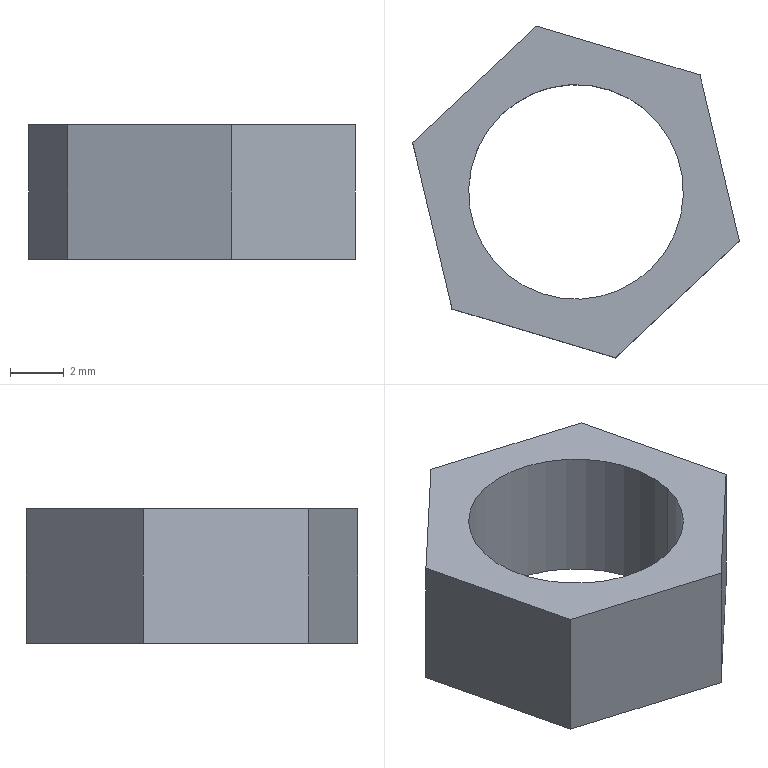Component | SolidWorks | 8Nut-1 | 1 solid | 10 faces | box 12.17 x 12.36 x 5 mm | volume 273 mm3 | plane 8 | cylinder 2 | commonest cylinder face diameters 8 x2
STEP:
#1=COLOUR_RGB('',0.7922,0.8196,0.9333);
#2=FILL_AREA_STYLE_COLOUR('',#1);
#3=FILL_AREA_STYLE('',(#2));
#4=SURFACE_STYLE_FILL_AREA(#3);
#5=SURFACE_SIDE_STYLE('',(#4));
#6=SURFACE_STYLE_USAGE(.BOTH.,#5);
#7=PRESENTATION_STYLE_ASSIGNMENT((#6));
#8=CARTESIAN_POINT('',(3.572,5.329,2.452));
#9=VERTEX_POINT('',#8);
#10=CARTESIAN_POINT('',(3.879,5.258,2.452));
#11=VERTEX_POINT('',#10);
#12=CARTESIAN_POINT('',(3.725,5.294,2.452));
#13=DIRECTION('',(0.,0.,1.));
#14=DIRECTION('',(0.9741,-0.2262,0.));
#15=AXIS2_PLACEMENT_3D('',#12,#13,#14);
#16=CIRCLE('',#15,0.1575);
#17=EDGE_CURVE('',#9,#11,#16,.T.);
#18=ORIENTED_EDGE('',*,*,#17,.T.);
#19=CARTESIAN_POINT('',(3.879,5.258,2.255));
#20=VERTEX_POINT('',#19);
#21=CARTESIAN_POINT('',(3.879,5.258,2.452));
#22=DIRECTION('',(0.,0.,-1.));
#23=VECTOR('',#22,39.37);
#24=LINE('',#21,#23);
#25=EDGE_CURVE('',#11,#20,#24,.T.);
#26=ORIENTED_EDGE('',*,*,#25,.T.);
#27=CARTESIAN_POINT('',(3.572,5.329,2.255));
#28=VERTEX_POINT('',#27);
#29=CARTESIAN_POINT('',(3.725,5.294,2.255));
#30=DIRECTION('',(0.,0.,1.));
#31=DIRECTION('',(0.9741,-0.2262,0.));
#32=AXIS2_PLACEMENT_3D('',#29,#30,#31);
#33=CIRCLE('',#32,0.1575);
#34=EDGE_CURVE('',#28,#20,#33,.T.);
#35=ORIENTED_EDGE('',*,*,#34,.F.);
#36=CARTESIAN_POINT('',(3.572,5.329,2.452));
#37=DIRECTION('',(0.,0.,-1.));
#38=VECTOR('',#37,39.37);
#39=LINE('',#36,#38);
#40=EDGE_CURVE('',#9,#28,#39,.T.);
#41=ORIENTED_EDGE('',*,*,#40,.F.);
#42=EDGE_LOOP('',(#18,#26,#35,#41));
#43=FACE_OUTER_BOUND('',#42,.T.);
#44=CARTESIAN_POINT('',(3.725,5.294,2.452));
#45=DIRECTION('',(0.,0.,-1.));
#46=DIRECTION('',(-0.9741,0.2262,0.));
#47=AXIS2_PLACEMENT_3D('',#44,#45,#46);
#48=CYLINDRICAL_SURFACE('',#47,0.1575);
#49=ADVANCED_FACE('',(#43),#48,.F.);
#50=CARTESIAN_POINT('',(3.907,5.465,2.452));
#51=VERTEX_POINT('',#50);
#52=CARTESIAN_POINT('',(3.668,5.537,2.452));
#53=VERTEX_POINT('',#52);
#54=CARTESIAN_POINT('',(3.907,5.465,2.452));
#55=DIRECTION('',(-0.9579,0.2872,0.));
#56=VECTOR('',#55,39.37);
#57=LINE('',#54,#56);
#58=EDGE_CURVE('',#51,#53,#57,.T.);
#59=ORIENTED_EDGE('',*,*,#58,.T.);
#60=CARTESIAN_POINT('',(3.486,5.366,2.452));
#61=VERTEX_POINT('',#60);
#62=CARTESIAN_POINT('',(3.668,5.537,2.452));
#63=DIRECTION('',(-0.7277,-0.6859,0.));
#64=VECTOR('',#63,39.37);
#65=LINE('',#62,#64);
#66=EDGE_CURVE('',#53,#61,#65,.T.);
#67=ORIENTED_EDGE('',*,*,#66,.T.);
#68=CARTESIAN_POINT('',(3.543,5.122,2.452));
#69=VERTEX_POINT('',#68);
#70=CARTESIAN_POINT('',(3.486,5.366,2.452));
#71=DIRECTION('',(0.2302,-0.9731,0.));
#72=VECTOR('',#71,39.37);
#73=LINE('',#70,#72);
#74=EDGE_CURVE('',#61,#69,#73,.T.);
#75=ORIENTED_EDGE('',*,*,#74,.T.);
#76=CARTESIAN_POINT('',(3.783,5.05,2.452));
#77=VERTEX_POINT('',#76);
#78=CARTESIAN_POINT('',(3.543,5.122,2.452));
#79=DIRECTION('',(0.9579,-0.2872,0.));
#80=VECTOR('',#79,39.37);
#81=LINE('',#78,#80);
#82=EDGE_CURVE('',#69,#77,#81,.T.);
#83=ORIENTED_EDGE('',*,*,#82,.T.);
#84=CARTESIAN_POINT('',(3.965,5.222,2.452));
#85=VERTEX_POINT('',#84);
#86=CARTESIAN_POINT('',(3.783,5.05,2.452));
#87=DIRECTION('',(0.7277,0.6859,0.));
#88=VECTOR('',#87,39.37);
#89=LINE('',#86,#88);
#90=EDGE_CURVE('',#77,#85,#89,.T.);
#91=ORIENTED_EDGE('',*,*,#90,.T.);
#92=CARTESIAN_POINT('',(3.965,5.222,2.452));
#93=DIRECTION('',(-0.2302,0.9731,0.));
#94=VECTOR('',#93,39.37);
#95=LINE('',#92,#94);
#96=EDGE_CURVE('',#85,#51,#95,.T.);
#97=ORIENTED_EDGE('',*,*,#96,.T.);
#98=EDGE_LOOP('',(#59,#67,#75,#83,#91,#97));
#99=FACE_OUTER_BOUND('',#98,.T.);
#100=ORIENTED_EDGE('',*,*,#17,.F.);
#101=CARTESIAN_POINT('',(3.725,5.294,2.452));
#102=DIRECTION('',(0.,0.,1.));
#103=DIRECTION('',(0.9741,-0.2262,0.));
#104=AXIS2_PLACEMENT_3D('',#101,#102,#103);
#105=CIRCLE('',#104,0.1575);
#106=EDGE_CURVE('',#11,#9,#105,.T.);
#107=ORIENTED_EDGE('',*,*,#106,.F.);
#108=EDGE_LOOP('',(#100,#107));
#109=FACE_BOUND('',#108,.T.);
#110=CARTESIAN_POINT('',(3.725,5.294,2.452));
#111=DIRECTION('',(0.,0.,1.));
#112=DIRECTION('',(0.9741,-0.2262,0.));
#113=AXIS2_PLACEMENT_3D('',#110,#111,#112);
#114=PLANE('',#113);
#115=ADVANCED_FACE('',(#99,#109),#114,.T.);
#116=CARTESIAN_POINT('',(3.907,5.465,2.255));
#117=VERTEX_POINT('',#116);
#118=CARTESIAN_POINT('',(3.668,5.537,2.255));
#119=VERTEX_POINT('',#118);
#120=CARTESIAN_POINT('',(3.907,5.465,2.255));
#121=DIRECTION('',(-0.9579,0.2872,0.));
#122=VECTOR('',#121,39.37);
#123=LINE('',#120,#122);
#124=EDGE_CURVE('',#117,#119,#123,.T.);
#125=ORIENTED_EDGE('',*,*,#124,.F.);
#126=CARTESIAN_POINT('',(3.965,5.222,2.255));
#127=VERTEX_POINT('',#126);
#128=CARTESIAN_POINT('',(3.965,5.222,2.255));
#129=DIRECTION('',(-0.2302,0.9731,0.));
#130=VECTOR('',#129,39.37);
#131=LINE('',#128,#130);
#132=EDGE_CURVE('',#127,#117,#131,.T.);
#133=ORIENTED_EDGE('',*,*,#132,.F.);
#134=CARTESIAN_POINT('',(3.783,5.05,2.255));
#135=VERTEX_POINT('',#134);
#136=CARTESIAN_POINT('',(3.783,5.05,2.255));
#137=DIRECTION('',(0.7277,0.6859,0.));
#138=VECTOR('',#137,39.37);
#139=LINE('',#136,#138);
#140=EDGE_CURVE('',#135,#127,#139,.T.);
#141=ORIENTED_EDGE('',*,*,#140,.F.);
#142=CARTESIAN_POINT('',(3.543,5.122,2.255));
#143=VERTEX_POINT('',#142);
#144=CARTESIAN_POINT('',(3.543,5.122,2.255));
#145=DIRECTION('',(0.9579,-0.2872,0.));
#146=VECTOR('',#145,39.37);
#147=LINE('',#144,#146);
#148=EDGE_CURVE('',#143,#135,#147,.T.);
#149=ORIENTED_EDGE('',*,*,#148,.F.);
#150=CARTESIAN_POINT('',(3.486,5.366,2.255));
#151=VERTEX_POINT('',#150);
#152=CARTESIAN_POINT('',(3.486,5.366,2.255));
#153=DIRECTION('',(0.2302,-0.9731,0.));
#154=VECTOR('',#153,39.37);
#155=LINE('',#152,#154);
#156=EDGE_CURVE('',#151,#143,#155,.T.);
#157=ORIENTED_EDGE('',*,*,#156,.F.);
#158=CARTESIAN_POINT('',(3.668,5.537,2.255));
#159=DIRECTION('',(-0.7277,-0.6859,0.));
#160=VECTOR('',#159,39.37);
#161=LINE('',#158,#160);
#162=EDGE_CURVE('',#119,#151,#161,.T.);
#163=ORIENTED_EDGE('',*,*,#162,.F.);
#164=EDGE_LOOP('',(#125,#133,#141,#149,#157,#163));
#165=FACE_OUTER_BOUND('',#164,.T.);
#166=ORIENTED_EDGE('',*,*,#34,.T.);
#167=CARTESIAN_POINT('',(3.725,5.294,2.255));
#168=DIRECTION('',(0.,0.,1.));
#169=DIRECTION('',(0.9741,-0.2262,0.));
#170=AXIS2_PLACEMENT_3D('',#167,#168,#169);
#171=CIRCLE('',#170,0.1575);
#172=EDGE_CURVE('',#20,#28,#171,.T.);
#173=ORIENTED_EDGE('',*,*,#172,.T.);
#174=EDGE_LOOP('',(#166,#173));
#175=FACE_BOUND('',#174,.T.);
#176=CARTESIAN_POINT('',(3.725,5.294,2.255));
#177=DIRECTION('',(0.,0.,1.));
#178=DIRECTION('',(0.9741,-0.2262,0.));
#179=AXIS2_PLACEMENT_3D('',#176,#177,#178);
#180=PLANE('',#179);
#181=ADVANCED_FACE('',(#165,#175),#180,.F.);
#182=ORIENTED_EDGE('',*,*,#124,.T.);
#183=CARTESIAN_POINT('',(3.668,5.537,2.452));
#184=DIRECTION('',(0.,0.,-1.));
#185=VECTOR('',#184,39.37);
#186=LINE('',#183,#185);
#187=EDGE_CURVE('',#53,#119,#186,.T.);
#188=ORIENTED_EDGE('',*,*,#187,.F.);
#189=ORIENTED_EDGE('',*,*,#58,.F.);
#190=CARTESIAN_POINT('',(3.907,5.465,2.452));
#191=DIRECTION('',(0.,0.,-1.));
#192=VECTOR('',#191,39.37);
#193=LINE('',#190,#192);
#194=EDGE_CURVE('',#51,#117,#193,.T.);
#195=ORIENTED_EDGE('',*,*,#194,.T.);
#196=EDGE_LOOP('',(#182,#188,#189,#195));
#197=FACE_OUTER_BOUND('',#196,.T.);
#198=CARTESIAN_POINT('',(3.907,5.465,2.452));
#199=DIRECTION('',(-0.2872,-0.9579,0.));
#200=DIRECTION('',(0.9579,-0.2872,0.));
#201=AXIS2_PLACEMENT_3D('',#198,#199,#200);
#202=PLANE('',#201);
#203=ADVANCED_FACE('',(#197),#202,.F.);
#204=ORIENTED_EDGE('',*,*,#162,.T.);
#205=CARTESIAN_POINT('',(3.486,5.366,2.452));
#206=DIRECTION('',(0.,0.,-1.));
#207=VECTOR('',#206,39.37);
#208=LINE('',#205,#207);
#209=EDGE_CURVE('',#61,#151,#208,.T.);
#210=ORIENTED_EDGE('',*,*,#209,.F.);
#211=ORIENTED_EDGE('',*,*,#66,.F.);
#212=ORIENTED_EDGE('',*,*,#187,.T.);
#213=EDGE_LOOP('',(#204,#210,#211,#212));
#214=FACE_OUTER_BOUND('',#213,.T.);
#215=CARTESIAN_POINT('',(3.668,5.537,2.452));
#216=DIRECTION('',(0.6859,-0.7277,0.));
#217=DIRECTION('',(0.7277,0.6859,0.));
#218=AXIS2_PLACEMENT_3D('',#215,#216,#217);
#219=PLANE('',#218);
#220=ADVANCED_FACE('',(#214),#219,.F.);
#221=ORIENTED_EDGE('',*,*,#156,.T.);
#222=CARTESIAN_POINT('',(3.543,5.122,2.452));
#223=DIRECTION('',(0.,0.,-1.));
#224=VECTOR('',#223,39.37);
#225=LINE('',#222,#224);
#226=EDGE_CURVE('',#69,#143,#225,.T.);
#227=ORIENTED_EDGE('',*,*,#226,.F.);
#228=ORIENTED_EDGE('',*,*,#74,.F.);
#229=ORIENTED_EDGE('',*,*,#209,.T.);
#230=EDGE_LOOP('',(#221,#227,#228,#229));
#231=FACE_OUTER_BOUND('',#230,.T.);
#232=CARTESIAN_POINT('',(3.486,5.366,2.452));
#233=DIRECTION('',(0.9731,0.2302,0.));
#234=DIRECTION('',(-0.2302,0.9731,0.));
#235=AXIS2_PLACEMENT_3D('',#232,#233,#234);
#236=PLANE('',#235);
#237=ADVANCED_FACE('',(#231),#236,.F.);
#238=ORIENTED_EDGE('',*,*,#148,.T.);
#239=CARTESIAN_POINT('',(3.783,5.05,2.452));
#240=DIRECTION('',(0.,0.,-1.));
#241=VECTOR('',#240,39.37);
#242=LINE('',#239,#241);
#243=EDGE_CURVE('',#77,#135,#242,.T.);
#244=ORIENTED_EDGE('',*,*,#243,.F.);
#245=ORIENTED_EDGE('',*,*,#82,.F.);
#246=ORIENTED_EDGE('',*,*,#226,.T.);
#247=EDGE_LOOP('',(#238,#244,#245,#246));
#248=FACE_OUTER_BOUND('',#247,.T.);
#249=CARTESIAN_POINT('',(3.543,5.122,2.452));
#250=DIRECTION('',(0.2872,0.9579,0.));
#251=DIRECTION('',(-0.9579,0.2872,0.));
#252=AXIS2_PLACEMENT_3D('',#249,#250,#251);
#253=PLANE('',#252);
#254=ADVANCED_FACE('',(#248),#253,.F.);
#255=ORIENTED_EDGE('',*,*,#140,.T.);
#256=CARTESIAN_POINT('',(3.965,5.222,2.452));
#257=DIRECTION('',(0.,0.,-1.));
#258=VECTOR('',#257,39.37);
#259=LINE('',#256,#258);
#260=EDGE_CURVE('',#85,#127,#259,.T.);
#261=ORIENTED_EDGE('',*,*,#260,.F.);
#262=ORIENTED_EDGE('',*,*,#90,.F.);
#263=ORIENTED_EDGE('',*,*,#243,.T.);
#264=EDGE_LOOP('',(#255,#261,#262,#263));
#265=FACE_OUTER_BOUND('',#264,.T.);
#266=CARTESIAN_POINT('',(3.783,5.05,2.452));
#267=DIRECTION('',(-0.6859,0.7277,0.));
#268=DIRECTION('',(-0.7277,-0.6859,0.));
#269=AXIS2_PLACEMENT_3D('',#266,#267,#268);
#270=PLANE('',#269);
#271=ADVANCED_FACE('',(#265),#270,.F.);
#272=ORIENTED_EDGE('',*,*,#132,.T.);
#273=ORIENTED_EDGE('',*,*,#194,.F.);
#274=ORIENTED_EDGE('',*,*,#96,.F.);
#275=ORIENTED_EDGE('',*,*,#260,.T.);
#276=EDGE_LOOP('',(#272,#273,#274,#275));
#277=FACE_OUTER_BOUND('',#276,.T.);
#278=CARTESIAN_POINT('',(3.965,5.222,2.452));
#279=DIRECTION('',(-0.9731,-0.2302,0.));
#280=DIRECTION('',(0.2302,-0.9731,0.));
#281=AXIS2_PLACEMENT_3D('',#278,#279,#280);
#282=PLANE('',#281);
#283=ADVANCED_FACE('',(#277),#282,.F.);
#284=ORIENTED_EDGE('',*,*,#25,.F.);
#285=ORIENTED_EDGE('',*,*,#106,.T.);
#286=ORIENTED_EDGE('',*,*,#40,.T.);
#287=ORIENTED_EDGE('',*,*,#172,.F.);
#288=EDGE_LOOP('',(#284,#285,#286,#287));
#289=FACE_OUTER_BOUND('',#288,.T.);
#290=CARTESIAN_POINT('',(3.725,5.294,2.452));
#291=DIRECTION('',(0.,0.,-1.));
#292=DIRECTION('',(-0.9741,0.2262,0.));
#293=AXIS2_PLACEMENT_3D('',#290,#291,#292);
#294=CYLINDRICAL_SURFACE('',#293,0.1575);
#295=ADVANCED_FACE('',(#289),#294,.F.);
#296=CLOSED_SHELL('',(#49,#115,#181,#203,#220,#237,#254,#271,#283,#295));
#297=MANIFOLD_SOLID_BREP('',#296);
#298=STYLED_ITEM('',(#7),#297);
#299=PRESENTATION_LAYER_ASSIGNMENT('','',(#298));
#300=CARTESIAN_POINT('',(0.,0.,0.));
#301=DIRECTION('',(0.,0.,1.));
#302=DIRECTION('',(1.,0.,0.));
#303=AXIS2_PLACEMENT_3D('',#300,#301,#302);
#304=(LENGTH_UNIT()NAMED_UNIT(*)SI_UNIT($,.METRE.));
#305=LENGTH_MEASURE_WITH_UNIT(LENGTH_MEASURE(0.0254),#304);
#306=DIMENSIONAL_EXPONENTS(1.,0.,0.,0.,0.,0.,0.);
#307=(CONVERSION_BASED_UNIT('',#305)LENGTH_UNIT()NAMED_UNIT(#306));
#308=UNCERTAINTY_MEASURE_WITH_UNIT(LENGTH_MEASURE(0.00001),#307,'','');
#309=(NAMED_UNIT(*)PLANE_ANGLE_UNIT()SI_UNIT($,.RADIAN.));
#310=(NAMED_UNIT(*)SI_UNIT($,.STERADIAN.)SOLID_ANGLE_UNIT());
#311=(GEOMETRIC_REPRESENTATION_CONTEXT(3)GLOBAL_UNCERTAINTY_ASSIGNED_CONTEXT((#308))GLOBAL_UNIT_ASSIGNED_CONTEXT((#307,#309,#310))REPRESENTATION_CONTEXT('',''));
#312=ADVANCED_BREP_SHAPE_REPRESENTATION('',(#297,#303),#311);
#313=(LENGTH_UNIT()NAMED_UNIT(*)SI_UNIT($,.METRE.));
#314=LENGTH_MEASURE_WITH_UNIT(LENGTH_MEASURE(0.0254),#313);
#315=DIMENSIONAL_EXPONENTS(1.,0.,0.,0.,0.,0.,0.);
#316=(CONVERSION_BASED_UNIT('',#314)LENGTH_UNIT()NAMED_UNIT(#315));
#317=UNCERTAINTY_MEASURE_WITH_UNIT(LENGTH_MEASURE(0.00001),#316,'','');
#318=(NAMED_UNIT(*)PLANE_ANGLE_UNIT()SI_UNIT($,.RADIAN.));
#319=(NAMED_UNIT(*)SI_UNIT($,.STERADIAN.)SOLID_ANGLE_UNIT());
#320=(GEOMETRIC_REPRESENTATION_CONTEXT(3)GLOBAL_UNCERTAINTY_ASSIGNED_CONTEXT((#317))GLOBAL_UNIT_ASSIGNED_CONTEXT((#316,#318,#319))REPRESENTATION_CONTEXT('',''));
#321=MECHANICAL_DESIGN_GEOMETRIC_PRESENTATION_REPRESENTATION('',(#298),#320);